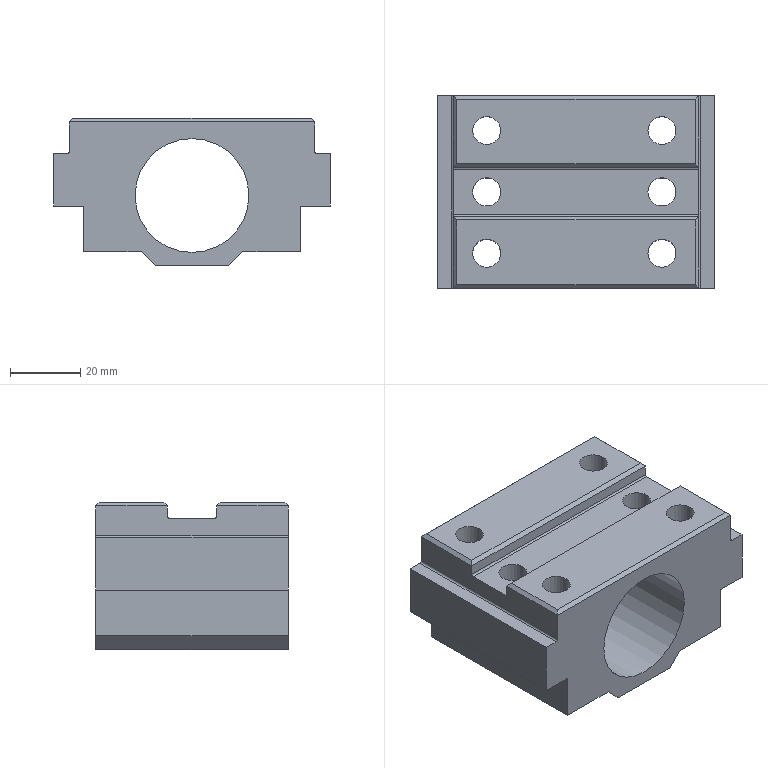Component | NX | MOVING_SLIDER | 1 solid | 49 faces | volume 91893 mm3 | plane 34 | cylinder 15 | commonest cylinder face diameters 8 x6 4 x4 1 x4 32.5 x1